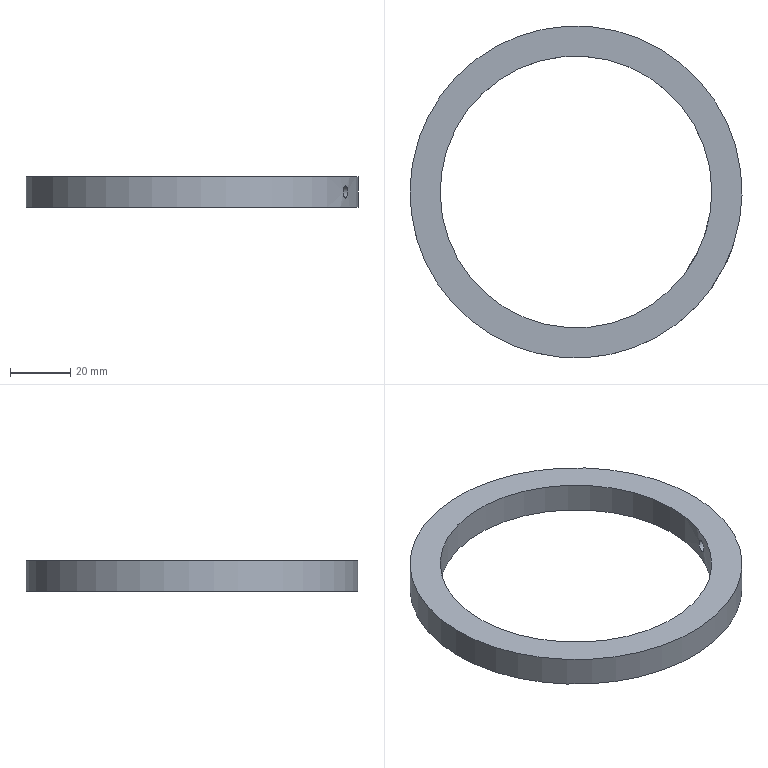Component | NX | CA6140-ZHUZHOU-ZHOUTAO3 | 1 solid | 5 faces | box 110 x 110 x 10 mm | volume 31291 mm3 | cylinder 3 | plane 2 | commonest cylinder face diameters 110 x1 90 x1 4 x1
STEP:
#1=CARTESIAN_POINT('',(0.,0.,0.));
#2=DIRECTION('',(0.,0.,1.));
#3=DIRECTION('',(1.,0.,0.));
#4=AXIS2_PLACEMENT_3D('',#1,#2,#3);
#5=CARTESIAN_POINT('',(17.204,41.581,-194.951));
#6=VERTEX_POINT('',#5);
#7=CARTESIAN_POINT('',(0.,-0.,-194.951));
#8=DIRECTION('',(0.,0.,-1.));
#9=DIRECTION('',(0.3823,0.924,0.));
#10=AXIS2_PLACEMENT_3D('',#7,#8,#9);
#11=CIRCLE('',#10,45.);
#12=CARTESIAN_POINT('',(0.,-0.,-194.951));
#13=DIRECTION('',(0.,0.,1.));
#14=DIRECTION('',(-0.3823,-0.924,0.));
#15=AXIS2_PLACEMENT_3D('',#12,#13,#14);
#16=PLANE('',#15);
#17=CARTESIAN_POINT('',(-45.,0.));
#18=CARTESIAN_POINT('',(-45.,77.942));
#19=CARTESIAN_POINT('',(22.5,38.971));
#20=CARTESIAN_POINT('',(90.,0.));
#21=CARTESIAN_POINT('',(22.5,-38.971));
#22=CARTESIAN_POINT('',(-45.,-77.942));
#23=CARTESIAN_POINT('',(-45.,0.));
#24=(BOUNDED_CURVE()B_SPLINE_CURVE(2,(#17,#18,#19,#20,#21,#22,#23),.UNSPECIFIED.,.T.,.F.)B_SPLINE_CURVE_WITH_KNOTS((1,2,2,2,2,1),(-2.094,0.,2.094,4.189,6.283,8.378),.UNSPECIFIED.)CURVE()GEOMETRIC_REPRESENTATION_ITEM()RATIONAL_B_SPLINE_CURVE((1.,0.5,1.,0.5,1.,0.5,1.))REPRESENTATION_ITEM(''));
#25=(GEOMETRIC_REPRESENTATION_CONTEXT(2)PARAMETRIC_REPRESENTATION_CONTEXT()REPRESENTATION_CONTEXT('',''));
#26=DEFINITIONAL_REPRESENTATION('',(#24),#25);
#27=PCURVE('',#16,#26);
#28=CARTESIAN_POINT('',(0.,-0.,-194.951));
#29=DIRECTION('',(0.,0.,-1.));
#30=DIRECTION('',(0.3823,0.924,0.));
#31=AXIS2_PLACEMENT_3D('',#28,#29,#30);
#32=CYLINDRICAL_SURFACE('',#31,45.);
#33=CARTESIAN_POINT('',(0.,0.));
#34=DIRECTION('',(1.,0.));
#35=VECTOR('',#34,1.);
#36=LINE('',#33,#35);
#37=(GEOMETRIC_REPRESENTATION_CONTEXT(2)PARAMETRIC_REPRESENTATION_CONTEXT()REPRESENTATION_CONTEXT('',''));
#38=DEFINITIONAL_REPRESENTATION('',(#36),#37);
#39=PCURVE('',#32,#38);
#40=SURFACE_CURVE('',#11,(#27,#39),.PCURVE_S1.);
#41=EDGE_CURVE('',#6,#6,#40,.T.);
#42=ORIENTED_EDGE('',*,*,#41,.T.);
#43=EDGE_LOOP('',(#42));
#44=FACE_BOUND('',#43,.T.);
#45=CARTESIAN_POINT('',(21.027,50.822,-194.951));
#46=VERTEX_POINT('',#45);
#47=CARTESIAN_POINT('',(-21.027,-50.822,-194.951));
#48=VERTEX_POINT('',#47);
#49=CARTESIAN_POINT('',(0.,-0.,-194.951));
#50=DIRECTION('',(0.,0.,-1.));
#51=DIRECTION('',(0.3823,0.924,0.));
#52=AXIS2_PLACEMENT_3D('',#49,#50,#51);
#53=CIRCLE('',#52,55.);
#54=CARTESIAN_POINT('',(-55.,0.));
#55=CARTESIAN_POINT('',(-55.,95.263));
#56=CARTESIAN_POINT('',(27.5,47.631));
#57=CARTESIAN_POINT('',(110.,0.));
#58=CARTESIAN_POINT('',(27.5,-47.631));
#59=CARTESIAN_POINT('',(-55.,-95.263));
#60=CARTESIAN_POINT('',(-55.,0.));
#61=(BOUNDED_CURVE()B_SPLINE_CURVE(2,(#54,#55,#56,#57,#58,#59,#60),.UNSPECIFIED.,.T.,.F.)B_SPLINE_CURVE_WITH_KNOTS((1,2,2,2,2,1),(-2.094,0.,2.094,4.189,6.283,8.378),.UNSPECIFIED.)CURVE()GEOMETRIC_REPRESENTATION_ITEM()RATIONAL_B_SPLINE_CURVE((1.,0.5,1.,0.5,1.,0.5,1.))REPRESENTATION_ITEM(''));
#62=(GEOMETRIC_REPRESENTATION_CONTEXT(2)PARAMETRIC_REPRESENTATION_CONTEXT()REPRESENTATION_CONTEXT('',''));
#63=DEFINITIONAL_REPRESENTATION('',(#61),#62);
#64=PCURVE('',#16,#63);
#65=CARTESIAN_POINT('',(0.,-0.,-204.951));
#66=DIRECTION('',(0.,0.,1.));
#67=DIRECTION('',(-0.3823,-0.924,0.));
#68=AXIS2_PLACEMENT_3D('',#65,#66,#67);
#69=CYLINDRICAL_SURFACE('',#68,55.);
#70=CARTESIAN_POINT('',(3.142,10.));
#71=DIRECTION('',(-1.,0.));
#72=VECTOR('',#71,1.);
#73=LINE('',#70,#72);
#74=(GEOMETRIC_REPRESENTATION_CONTEXT(2)PARAMETRIC_REPRESENTATION_CONTEXT()REPRESENTATION_CONTEXT('',''));
#75=DEFINITIONAL_REPRESENTATION('',(#73),#74);
#76=PCURVE('',#69,#75);
#77=SURFACE_CURVE('',#53,(#64,#76),.PCURVE_S1.);
#78=EDGE_CURVE('',#46,#48,#77,.T.);
#79=ORIENTED_EDGE('',*,*,#78,.F.);
#80=CARTESIAN_POINT('',(0.,-0.,-194.951));
#81=DIRECTION('',(0.,0.,-1.));
#82=DIRECTION('',(0.3823,0.924,0.));
#83=AXIS2_PLACEMENT_3D('',#80,#81,#82);
#84=CIRCLE('',#83,55.);
#85=CARTESIAN_POINT('',(-55.,0.));
#86=CARTESIAN_POINT('',(-55.,95.263));
#87=CARTESIAN_POINT('',(27.5,47.631));
#88=CARTESIAN_POINT('',(110.,0.));
#89=CARTESIAN_POINT('',(27.5,-47.631));
#90=CARTESIAN_POINT('',(-55.,-95.263));
#91=CARTESIAN_POINT('',(-55.,0.));
#92=(BOUNDED_CURVE()B_SPLINE_CURVE(2,(#85,#86,#87,#88,#89,#90,#91),.UNSPECIFIED.,.T.,.F.)B_SPLINE_CURVE_WITH_KNOTS((1,2,2,2,2,1),(-2.094,0.,2.094,4.189,6.283,8.378),.UNSPECIFIED.)CURVE()GEOMETRIC_REPRESENTATION_ITEM()RATIONAL_B_SPLINE_CURVE((1.,0.5,1.,0.5,1.,0.5,1.))REPRESENTATION_ITEM(''));
#93=(GEOMETRIC_REPRESENTATION_CONTEXT(2)PARAMETRIC_REPRESENTATION_CONTEXT()REPRESENTATION_CONTEXT('',''));
#94=DEFINITIONAL_REPRESENTATION('',(#92),#93);
#95=PCURVE('',#16,#94);
#96=CARTESIAN_POINT('',(9.425,10.));
#97=DIRECTION('',(-1.,0.));
#98=VECTOR('',#97,1.);
#99=LINE('',#96,#98);
#100=(GEOMETRIC_REPRESENTATION_CONTEXT(2)PARAMETRIC_REPRESENTATION_CONTEXT()REPRESENTATION_CONTEXT('',''));
#101=DEFINITIONAL_REPRESENTATION('',(#99),#100);
#102=PCURVE('',#69,#101);
#103=SURFACE_CURVE('',#84,(#95,#102),.PCURVE_S1.);
#104=EDGE_CURVE('',#48,#46,#103,.T.);
#105=ORIENTED_EDGE('',*,*,#104,.F.);
#106=EDGE_LOOP('',(#79,#105));
#107=FACE_BOUND('',#106,.T.);
#108=ADVANCED_FACE('',(#44,#107),#16,.T.);
#109=CARTESIAN_POINT('',(17.204,41.581,-204.951));
#110=VERTEX_POINT('',#109);
#111=CARTESIAN_POINT('',(0.,-0.,-204.951));
#112=DIRECTION('',(0.,0.,-1.));
#113=DIRECTION('',(0.3823,0.924,0.));
#114=AXIS2_PLACEMENT_3D('',#111,#112,#113);
#115=CIRCLE('',#114,45.);
#116=CARTESIAN_POINT('',(0.,-0.,-204.951));
#117=DIRECTION('',(0.,0.,-1.));
#118=DIRECTION('',(0.3823,0.924,0.));
#119=AXIS2_PLACEMENT_3D('',#116,#117,#118);
#120=PLANE('',#119);
#121=CARTESIAN_POINT('',(0.,0.));
#122=DIRECTION('',(1.,0.));
#123=AXIS2_PLACEMENT_2D('',#121,#122);
#124=CIRCLE('',#123,45.);
#125=(GEOMETRIC_REPRESENTATION_CONTEXT(2)PARAMETRIC_REPRESENTATION_CONTEXT()REPRESENTATION_CONTEXT('',''));
#126=DEFINITIONAL_REPRESENTATION('',(#124),#125);
#127=PCURVE('',#120,#126);
#128=CARTESIAN_POINT('',(0.,10.));
#129=DIRECTION('',(1.,0.));
#130=VECTOR('',#129,1.);
#131=LINE('',#128,#130);
#132=(GEOMETRIC_REPRESENTATION_CONTEXT(2)PARAMETRIC_REPRESENTATION_CONTEXT()REPRESENTATION_CONTEXT('',''));
#133=DEFINITIONAL_REPRESENTATION('',(#131),#132);
#134=PCURVE('',#32,#133);
#135=SURFACE_CURVE('',#115,(#127,#134),.PCURVE_S1.);
#136=EDGE_CURVE('',#110,#110,#135,.T.);
#137=ORIENTED_EDGE('',*,*,#136,.F.);
#138=EDGE_LOOP('',(#137));
#139=FACE_BOUND('',#138,.T.);
#140=CARTESIAN_POINT('',(-21.027,-50.822,-204.951));
#141=VERTEX_POINT('',#140);
#142=CARTESIAN_POINT('',(0.,-0.,-204.951));
#143=DIRECTION('',(0.,0.,1.));
#144=DIRECTION('',(-0.3823,-0.924,0.));
#145=AXIS2_PLACEMENT_3D('',#142,#143,#144);
#146=CIRCLE('',#145,55.);
#147=CARTESIAN_POINT('',(-55.,0.));
#148=CARTESIAN_POINT('',(-55.,95.263));
#149=CARTESIAN_POINT('',(27.5,47.631));
#150=CARTESIAN_POINT('',(110.,0.));
#151=CARTESIAN_POINT('',(27.5,-47.631));
#152=CARTESIAN_POINT('',(-55.,-95.263));
#153=CARTESIAN_POINT('',(-55.,0.));
#154=(BOUNDED_CURVE()B_SPLINE_CURVE(2,(#147,#148,#149,#150,#151,#152,#153),.UNSPECIFIED.,.T.,.F.)B_SPLINE_CURVE_WITH_KNOTS((1,2,2,2,2,1),(-2.094,0.,2.094,4.189,6.283,8.378),.UNSPECIFIED.)CURVE()GEOMETRIC_REPRESENTATION_ITEM()RATIONAL_B_SPLINE_CURVE((1.,0.5,1.,0.5,1.,0.5,1.))REPRESENTATION_ITEM(''));
#155=(GEOMETRIC_REPRESENTATION_CONTEXT(2)PARAMETRIC_REPRESENTATION_CONTEXT()REPRESENTATION_CONTEXT('',''));
#156=DEFINITIONAL_REPRESENTATION('',(#154),#155);
#157=PCURVE('',#120,#156);
#158=CARTESIAN_POINT('',(0.,0.));
#159=DIRECTION('',(1.,0.));
#160=VECTOR('',#159,1.);
#161=LINE('',#158,#160);
#162=(GEOMETRIC_REPRESENTATION_CONTEXT(2)PARAMETRIC_REPRESENTATION_CONTEXT()REPRESENTATION_CONTEXT('',''));
#163=DEFINITIONAL_REPRESENTATION('',(#161),#162);
#164=PCURVE('',#69,#163);
#165=SURFACE_CURVE('',#146,(#157,#164),.PCURVE_S1.);
#166=EDGE_CURVE('',#141,#141,#165,.T.);
#167=ORIENTED_EDGE('',*,*,#166,.F.);
#168=EDGE_LOOP('',(#167));
#169=FACE_BOUND('',#168,.T.);
#170=ADVANCED_FACE('',(#139,#169),#120,.T.);
#171=ORIENTED_EDGE('',*,*,#78,.T.);
#172=CARTESIAN_POINT('',(-21.027,-50.822,-204.951));
#173=CARTESIAN_POINT('',(-21.027,-50.822,-194.951));
#174=B_SPLINE_CURVE_WITH_KNOTS('',1,(#172,#173),.UNSPECIFIED.,.F.,.F.,(2,2),(0.,10.),.PIECEWISE_BEZIER_KNOTS.);
#175=CARTESIAN_POINT('',(0.,0.));
#176=DIRECTION('',(0.,1.));
#177=VECTOR('',#176,1.);
#178=LINE('',#175,#177);
#179=(GEOMETRIC_REPRESENTATION_CONTEXT(2)PARAMETRIC_REPRESENTATION_CONTEXT()REPRESENTATION_CONTEXT('',''));
#180=DEFINITIONAL_REPRESENTATION('',(#178),#179);
#181=PCURVE('',#69,#180);
#182=CARTESIAN_POINT('',(6.283,0.));
#183=DIRECTION('',(0.,1.));
#184=VECTOR('',#183,1.);
#185=LINE('',#182,#184);
#186=(GEOMETRIC_REPRESENTATION_CONTEXT(2)PARAMETRIC_REPRESENTATION_CONTEXT()REPRESENTATION_CONTEXT('',''));
#187=DEFINITIONAL_REPRESENTATION('',(#185),#186);
#188=PCURVE('',#69,#187);
#189=SEAM_CURVE('',#174,(#181,#188),.PCURVE_S1.);
#190=EDGE_CURVE('',#141,#48,#189,.T.);
#191=ORIENTED_EDGE('',*,*,#190,.F.);
#192=ORIENTED_EDGE('',*,*,#166,.T.);
#193=ORIENTED_EDGE('',*,*,#190,.T.);
#194=ORIENTED_EDGE('',*,*,#104,.T.);
#195=EDGE_LOOP('',(#171,#191,#192,#193,#194));
#196=FACE_BOUND('',#195,.T.);
#197=CARTESIAN_POINT('',(50.822,-21.027,-201.951));
#198=VERTEX_POINT('',#197);
#199=CARTESIAN_POINT('',(50.822,-21.027,-201.951));
#200=CARTESIAN_POINT('',(50.907,-20.821,-201.951));
#201=CARTESIAN_POINT('',(50.993,-20.611,-201.912));
#202=CARTESIAN_POINT('',(51.071,-20.414,-201.838));
#203=CARTESIAN_POINT('',(51.149,-20.218,-201.764));
#204=CARTESIAN_POINT('',(51.223,-20.031,-201.653));
#205=CARTESIAN_POINT('',(51.286,-19.868,-201.513));
#206=CARTESIAN_POINT('',(51.349,-19.705,-201.373));
#207=CARTESIAN_POINT('',(51.404,-19.562,-201.201));
#208=CARTESIAN_POINT('',(51.446,-19.451,-201.011));
#209=CARTESIAN_POINT('',(51.488,-19.34,-200.822));
#210=CARTESIAN_POINT('',(51.518,-19.258,-200.609));
#211=CARTESIAN_POINT('',(51.536,-19.211,-200.39));
#212=CARTESIAN_POINT('',(51.553,-19.165,-200.172));
#213=CARTESIAN_POINT('',(51.557,-19.154,-199.942));
#214=CARTESIAN_POINT('',(51.548,-19.178,-199.72));
#215=CARTESIAN_POINT('',(51.539,-19.202,-199.498));
#216=CARTESIAN_POINT('',(51.517,-19.263,-199.277));
#217=CARTESIAN_POINT('',(51.482,-19.354,-199.076));
#218=CARTESIAN_POINT('',(51.448,-19.446,-198.874));
#219=CARTESIAN_POINT('',(51.4,-19.572,-198.687));
#220=CARTESIAN_POINT('',(51.343,-19.72,-198.53));
#221=CARTESIAN_POINT('',(51.286,-19.868,-198.372));
#222=CARTESIAN_POINT('',(51.218,-20.044,-198.24));
#223=CARTESIAN_POINT('',(51.144,-20.232,-198.144));
#224=CARTESIAN_POINT('',(51.069,-20.42,-198.048));
#225=CARTESIAN_POINT('',(50.986,-20.626,-197.986));
#226=CARTESIAN_POINT('',(50.902,-20.832,-197.962));
#227=CARTESIAN_POINT('',(50.818,-21.038,-197.938));
#228=CARTESIAN_POINT('',(50.73,-21.25,-197.953));
#229=CARTESIAN_POINT('',(50.645,-21.45,-198.004));
#230=CARTESIAN_POINT('',(50.56,-21.651,-198.055));
#231=CARTESIAN_POINT('',(50.476,-21.846,-198.145));
#232=CARTESIAN_POINT('',(50.4,-22.018,-198.265));
#233=CARTESIAN_POINT('',(50.325,-22.191,-198.386));
#234=CARTESIAN_POINT('',(50.256,-22.347,-198.54));
#235=CARTESIAN_POINT('',(50.199,-22.473,-198.716));
#236=CARTESIAN_POINT('',(50.143,-22.599,-198.893));
#237=CARTESIAN_POINT('',(50.097,-22.699,-199.095));
#238=CARTESIAN_POINT('',(50.068,-22.765,-199.307));
#239=CARTESIAN_POINT('',(50.038,-22.83,-199.519));
#240=CARTESIAN_POINT('',(50.023,-22.864,-199.746));
#241=CARTESIAN_POINT('',(50.023,-22.862,-199.97));
#242=CARTESIAN_POINT('',(50.024,-22.86,-200.194));
#243=CARTESIAN_POINT('',(50.041,-22.822,-200.42));
#244=CARTESIAN_POINT('',(50.073,-22.753,-200.631));
#245=CARTESIAN_POINT('',(50.104,-22.684,-200.841));
#246=CARTESIAN_POINT('',(50.151,-22.58,-201.041));
#247=CARTESIAN_POINT('',(50.209,-22.451,-201.215));
#248=CARTESIAN_POINT('',(50.267,-22.322,-201.388));
#249=CARTESIAN_POINT('',(50.337,-22.164,-201.54));
#250=CARTESIAN_POINT('',(50.413,-21.989,-201.656));
#251=CARTESIAN_POINT('',(50.49,-21.814,-201.773));
#252=CARTESIAN_POINT('',(50.574,-21.617,-201.859));
#253=CARTESIAN_POINT('',(50.659,-21.416,-201.906));
#254=CARTESIAN_POINT('',(50.713,-21.289,-201.936));
#255=CARTESIAN_POINT('',(50.768,-21.158,-201.951));
#256=CARTESIAN_POINT('',(50.822,-21.027,-201.951));
#257=B_SPLINE_CURVE_WITH_KNOTS('',3,(#199,#200,#201,#202,#203,#204,#205,#206,#207,#208,#209,#210,#211,#212,#213,#214,#215,#216,#217,#218,#219,#220,#221,#222,#223,#224,#225,#226,#227,#228,#229,#230,#231,#232,#233,#234,#235,#236,#237,#238,#239,#240,#241,#242,#243,#244,#245,#246,#247,#248,#249,#250,#251,#252,#253,#254,#255,#256),.UNSPECIFIED.,.T.,.F.,(1,3,3,3,3,3,3,3,3,3,3,3,3,3,3,3,3,3,3,3,3,1),(-0.03354,0.,0.05368,0.1074,0.1611,0.2148,0.2685,0.3221,0.3758,0.4295,0.4832,0.5369,0.5906,0.6443,0.698,0.7517,0.8054,0.859,0.9127,0.9665,1.,1.054),.UNSPECIFIED.);
#258=CARTESIAN_POINT('',(1.571,3.));
#259=CARTESIAN_POINT('',(1.572,3.));
#260=CARTESIAN_POINT('',(1.573,3.003));
#261=CARTESIAN_POINT('',(1.576,3.019));
#262=CARTESIAN_POINT('',(1.579,3.044));
#263=CARTESIAN_POINT('',(1.581,3.08));
#264=CARTESIAN_POINT('',(1.584,3.124));
#265=CARTESIAN_POINT('',(1.586,3.179));
#266=CARTESIAN_POINT('',(1.588,3.243));
#267=CARTESIAN_POINT('',(1.59,3.316));
#268=CARTESIAN_POINT('',(1.593,3.398));
#269=CARTESIAN_POINT('',(1.595,3.487));
#270=CARTESIAN_POINT('',(1.597,3.584));
#271=CARTESIAN_POINT('',(1.598,3.689));
#272=CARTESIAN_POINT('',(1.6,3.801));
#273=CARTESIAN_POINT('',(1.601,3.918));
#274=CARTESIAN_POINT('',(1.603,4.04));
#275=CARTESIAN_POINT('',(1.604,4.168));
#276=CARTESIAN_POINT('',(1.605,4.3));
#277=CARTESIAN_POINT('',(1.606,4.436));
#278=CARTESIAN_POINT('',(1.606,4.574));
#279=CARTESIAN_POINT('',(1.607,4.714));
#280=CARTESIAN_POINT('',(1.607,4.857));
#281=CARTESIAN_POINT('',(1.607,5.));
#282=CARTESIAN_POINT('',(1.607,5.143));
#283=CARTESIAN_POINT('',(1.607,5.284));
#284=CARTESIAN_POINT('',(1.606,5.424));
#285=CARTESIAN_POINT('',(1.606,5.563));
#286=CARTESIAN_POINT('',(1.605,5.699));
#287=CARTESIAN_POINT('',(1.604,5.831));
#288=CARTESIAN_POINT('',(1.603,5.958));
#289=CARTESIAN_POINT('',(1.601,6.081));
#290=CARTESIAN_POINT('',(1.6,6.199));
#291=CARTESIAN_POINT('',(1.598,6.31));
#292=CARTESIAN_POINT('',(1.597,6.415));
#293=CARTESIAN_POINT('',(1.595,6.512));
#294=CARTESIAN_POINT('',(1.593,6.602));
#295=CARTESIAN_POINT('',(1.59,6.683));
#296=CARTESIAN_POINT('',(1.588,6.757));
#297=CARTESIAN_POINT('',(1.586,6.82));
#298=CARTESIAN_POINT('',(1.584,6.875));
#299=CARTESIAN_POINT('',(1.581,6.92));
#300=CARTESIAN_POINT('',(1.579,6.956));
#301=CARTESIAN_POINT('',(1.576,6.981));
#302=CARTESIAN_POINT('',(1.573,6.996));
#303=CARTESIAN_POINT('',(1.571,7.002));
#304=CARTESIAN_POINT('',(1.568,6.996));
#305=CARTESIAN_POINT('',(1.566,6.981));
#306=CARTESIAN_POINT('',(1.563,6.956));
#307=CARTESIAN_POINT('',(1.561,6.921));
#308=CARTESIAN_POINT('',(1.558,6.876));
#309=CARTESIAN_POINT('',(1.556,6.821));
#310=CARTESIAN_POINT('',(1.553,6.757));
#311=CARTESIAN_POINT('',(1.551,6.685));
#312=CARTESIAN_POINT('',(1.549,6.603));
#313=CARTESIAN_POINT('',(1.547,6.514));
#314=CARTESIAN_POINT('',(1.545,6.416));
#315=CARTESIAN_POINT('',(1.543,6.312));
#316=CARTESIAN_POINT('',(1.542,6.201));
#317=CARTESIAN_POINT('',(1.54,6.084));
#318=CARTESIAN_POINT('',(1.539,5.961));
#319=CARTESIAN_POINT('',(1.538,5.833));
#320=CARTESIAN_POINT('',(1.537,5.701));
#321=CARTESIAN_POINT('',(1.536,5.566));
#322=CARTESIAN_POINT('',(1.535,5.427));
#323=CARTESIAN_POINT('',(1.535,5.287));
#324=CARTESIAN_POINT('',(1.534,5.144));
#325=CARTESIAN_POINT('',(1.534,5.002));
#326=CARTESIAN_POINT('',(1.534,4.86));
#327=CARTESIAN_POINT('',(1.535,4.717));
#328=CARTESIAN_POINT('',(1.535,4.576));
#329=CARTESIAN_POINT('',(1.536,4.437));
#330=CARTESIAN_POINT('',(1.537,4.302));
#331=CARTESIAN_POINT('',(1.538,4.171));
#332=CARTESIAN_POINT('',(1.539,4.043));
#333=CARTESIAN_POINT('',(1.54,3.919));
#334=CARTESIAN_POINT('',(1.542,3.802));
#335=CARTESIAN_POINT('',(1.543,3.691));
#336=CARTESIAN_POINT('',(1.545,3.586));
#337=CARTESIAN_POINT('',(1.547,3.489));
#338=CARTESIAN_POINT('',(1.549,3.399));
#339=CARTESIAN_POINT('',(1.551,3.317));
#340=CARTESIAN_POINT('',(1.553,3.244));
#341=CARTESIAN_POINT('',(1.556,3.18));
#342=CARTESIAN_POINT('',(1.558,3.125));
#343=CARTESIAN_POINT('',(1.561,3.08));
#344=CARTESIAN_POINT('',(1.563,3.045));
#345=CARTESIAN_POINT('',(1.566,3.019));
#346=CARTESIAN_POINT('',(1.568,3.003));
#347=CARTESIAN_POINT('',(1.57,3.));
#348=CARTESIAN_POINT('',(1.571,3.));
#349=B_SPLINE_CURVE_WITH_KNOTS('',3,(#258,#259,#260,#261,#262,#263,#264,#265,#266,#267,#268,#269,#270,#271,#272,#273,#274,#275,#276,#277,#278,#279,#280,#281,#282,#283,#284,#285,#286,#287,#288,#289,#290,#291,#292,#293,#294,#295,#296,#297,#298,#299,#300,#301,#302,#303,#304,#305,#306,#307,#308,#309,#310,#311,#312,#313,#314,#315,#316,#317,#318,#319,#320,#321,#322,#323,#324,#325,#326,#327,#328,#329,#330,#331,#332,#333,#334,#335,#336,#337,#338,#339,#340,#341,#342,#343,#344,#345,#346,#347,#348),.UNSPECIFIED.,.T.,.F.,(4,1,1,1,1,1,1,1,1,1,1,1,1,1,1,1,1,1,1,1,1,1,1,1,1,1,1,1,1,1,1,1,1,1,1,1,1,1,1,1,1,1,1,1,1,1,1,1,1,1,1,1,1,1,1,1,1,1,1,1,1,1,1,1,1,1,1,1,1,1,1,1,1,1,1,1,1,1,1,1,1,1,1,1,1,1,1,1,4),(0.,0.01136,0.02273,0.03409,0.04545,0.05682,0.06818,0.07955,0.09091,0.1023,0.1136,0.125,0.1364,0.1477,0.1591,0.1705,0.1818,0.1932,0.2045,0.2159,0.2273,0.2386,0.25,0.2614,0.2727,0.2841,0.2955,0.3068,0.3182,0.3295,0.3409,0.3523,0.3636,0.375,0.3864,0.3977,0.4091,0.4205,0.4318,0.4432,0.4545,0.4659,0.4773,0.4886,0.5,0.5114,0.5227,0.5341,0.5455,0.5568,0.5682,0.5795,0.5909,0.6023,0.6136,0.625,0.6364,0.6477,0.6591,0.6705,0.6818,0.6932,0.7045,0.7159,0.7273,0.7386,0.75,0.7614,0.7727,0.7841,0.7955,0.8068,0.8182,0.8295,0.8409,0.8523,0.8636,0.875,0.8864,0.8977,0.9091,0.9205,0.9318,0.9432,0.9545,0.9659,0.9773,0.9886,1.),.QUASI_UNIFORM_KNOTS.);
#350=(GEOMETRIC_REPRESENTATION_CONTEXT(2)PARAMETRIC_REPRESENTATION_CONTEXT()REPRESENTATION_CONTEXT('',''));
#351=DEFINITIONAL_REPRESENTATION('',(#349),#350);
#352=PCURVE('',#69,#351);
#353=CARTESIAN_POINT('',(55.442,-22.939,-199.951));
#354=DIRECTION('',(-0.924,0.3823,0.));
#355=DIRECTION('',(0.,0.,-1.));
#356=AXIS2_PLACEMENT_3D('',#353,#354,#355);
#357=CYLINDRICAL_SURFACE('',#356,2.);
#358=CARTESIAN_POINT('',(6.283,5.));
#359=CARTESIAN_POINT('',(0.,5.));
#360=B_SPLINE_CURVE_WITH_KNOTS('',1,(#358,#359),.UNSPECIFIED.,.F.,.F.,(2,2),(0.,1.),.PIECEWISE_BEZIER_KNOTS.);
#361=(GEOMETRIC_REPRESENTATION_CONTEXT(2)PARAMETRIC_REPRESENTATION_CONTEXT()REPRESENTATION_CONTEXT('',''));
#362=DEFINITIONAL_REPRESENTATION('',(#360),#361);
#363=PCURVE('',#357,#362);
#364=SURFACE_CURVE('',#257,(#352,#363),.PCURVE_S1.);
#365=EDGE_CURVE('',#198,#198,#364,.T.);
#366=ORIENTED_EDGE('',*,*,#365,.F.);
#367=EDGE_LOOP('',(#366));
#368=FACE_BOUND('',#367,.T.);
#369=ADVANCED_FACE('',(#196,#368),#69,.T.);
#370=ORIENTED_EDGE('',*,*,#136,.F.);
#371=CARTESIAN_POINT('',(17.204,41.581,-194.951));
#372=CARTESIAN_POINT('',(17.204,41.581,-204.951));
#373=B_SPLINE_CURVE_WITH_KNOTS('',1,(#371,#372),.UNSPECIFIED.,.F.,.F.,(2,2),(0.,10.),.PIECEWISE_BEZIER_KNOTS.);
#374=CARTESIAN_POINT('',(0.,0.));
#375=DIRECTION('',(0.,1.));
#376=VECTOR('',#375,1.);
#377=LINE('',#374,#376);
#378=(GEOMETRIC_REPRESENTATION_CONTEXT(2)PARAMETRIC_REPRESENTATION_CONTEXT()REPRESENTATION_CONTEXT('',''));
#379=DEFINITIONAL_REPRESENTATION('',(#377),#378);
#380=PCURVE('',#32,#379);
#381=CARTESIAN_POINT('',(6.283,0.));
#382=DIRECTION('',(0.,1.));
#383=VECTOR('',#382,1.);
#384=LINE('',#381,#383);
#385=(GEOMETRIC_REPRESENTATION_CONTEXT(2)PARAMETRIC_REPRESENTATION_CONTEXT()REPRESENTATION_CONTEXT('',''));
#386=DEFINITIONAL_REPRESENTATION('',(#384),#385);
#387=PCURVE('',#32,#386);
#388=SEAM_CURVE('',#373,(#380,#387),.PCURVE_S1.);
#389=EDGE_CURVE('',#6,#110,#388,.T.);
#390=ORIENTED_EDGE('',*,*,#389,.F.);
#391=ORIENTED_EDGE('',*,*,#41,.T.);
#392=ORIENTED_EDGE('',*,*,#389,.T.);
#393=EDGE_LOOP('',(#370,#390,#391,#392));
#394=FACE_BOUND('',#393,.F.);
#395=CARTESIAN_POINT('',(41.581,-17.204,-201.951));
#396=VERTEX_POINT('',#395);
#397=CARTESIAN_POINT('',(41.581,-17.204,-201.951));
#398=CARTESIAN_POINT('',(41.667,-16.998,-201.951));
#399=CARTESIAN_POINT('',(41.752,-16.787,-201.912));
#400=CARTESIAN_POINT('',(41.83,-16.591,-201.838));
#401=CARTESIAN_POINT('',(41.908,-16.395,-201.764));
#402=CARTESIAN_POINT('',(41.98,-16.207,-201.653));
#403=CARTESIAN_POINT('',(42.043,-16.044,-201.513));
#404=CARTESIAN_POINT('',(42.105,-15.88,-201.373));
#405=CARTESIAN_POINT('',(42.159,-15.737,-201.201));
#406=CARTESIAN_POINT('',(42.2,-15.626,-201.012));
#407=CARTESIAN_POINT('',(42.241,-15.514,-200.822));
#408=CARTESIAN_POINT('',(42.271,-15.432,-200.609));
#409=CARTESIAN_POINT('',(42.288,-15.385,-200.391));
#410=CARTESIAN_POINT('',(42.305,-15.339,-200.172));
#411=CARTESIAN_POINT('',(42.309,-15.328,-199.942));
#412=CARTESIAN_POINT('',(42.3,-15.352,-199.72));
#413=CARTESIAN_POINT('',(42.292,-15.376,-199.498));
#414=CARTESIAN_POINT('',(42.27,-15.437,-199.277));
#415=CARTESIAN_POINT('',(42.236,-15.529,-199.076));
#416=CARTESIAN_POINT('',(42.202,-15.62,-198.875));
#417=CARTESIAN_POINT('',(42.156,-15.746,-198.688));
#418=CARTESIAN_POINT('',(42.099,-15.895,-198.53));
#419=CARTESIAN_POINT('',(42.043,-16.044,-198.373));
#420=CARTESIAN_POINT('',(41.976,-16.22,-198.24));
#421=CARTESIAN_POINT('',(41.902,-16.408,-198.144));
#422=CARTESIAN_POINT('',(41.828,-16.596,-198.048));
#423=CARTESIAN_POINT('',(41.746,-16.802,-197.986));
#424=CARTESIAN_POINT('',(41.662,-17.008,-197.962));
#425=CARTESIAN_POINT('',(41.578,-17.214,-197.938));
#426=CARTESIAN_POINT('',(41.49,-17.426,-197.953));
#427=CARTESIAN_POINT('',(41.404,-17.626,-198.004));
#428=CARTESIAN_POINT('',(41.319,-17.827,-198.055));
#429=CARTESIAN_POINT('',(41.234,-18.021,-198.144));
#430=CARTESIAN_POINT('',(41.158,-18.193,-198.265));
#431=CARTESIAN_POINT('',(41.082,-18.366,-198.385));
#432=CARTESIAN_POINT('',(41.012,-18.522,-198.54));
#433=CARTESIAN_POINT('',(40.955,-18.647,-198.716));
#434=CARTESIAN_POINT('',(40.897,-18.773,-198.892));
#435=CARTESIAN_POINT('',(40.851,-18.873,-199.094));
#436=CARTESIAN_POINT('',(40.821,-18.939,-199.306));
#437=CARTESIAN_POINT('',(40.79,-19.004,-199.518));
#438=CARTESIAN_POINT('',(40.775,-19.037,-199.745));
#439=CARTESIAN_POINT('',(40.776,-19.035,-199.969));
#440=CARTESIAN_POINT('',(40.777,-19.033,-200.193));
#441=CARTESIAN_POINT('',(40.794,-18.997,-200.419));
#442=CARTESIAN_POINT('',(40.826,-18.928,-200.63));
#443=CARTESIAN_POINT('',(40.858,-18.859,-200.84));
#444=CARTESIAN_POINT('',(40.905,-18.756,-201.04));
#445=CARTESIAN_POINT('',(40.964,-18.627,-201.214));
#446=CARTESIAN_POINT('',(41.022,-18.498,-201.387));
#447=CARTESIAN_POINT('',(41.093,-18.34,-201.539));
#448=CARTESIAN_POINT('',(41.17,-18.166,-201.656));
#449=CARTESIAN_POINT('',(41.247,-17.991,-201.773));
#450=CARTESIAN_POINT('',(41.333,-17.795,-201.858));
#451=CARTESIAN_POINT('',(41.418,-17.594,-201.906));
#452=CARTESIAN_POINT('',(41.472,-17.466,-201.936));
#453=CARTESIAN_POINT('',(41.527,-17.335,-201.951));
#454=CARTESIAN_POINT('',(41.581,-17.204,-201.951));
#455=B_SPLINE_CURVE_WITH_KNOTS('',3,(#397,#398,#399,#400,#401,#402,#403,#404,#405,#406,#407,#408,#409,#410,#411,#412,#413,#414,#415,#416,#417,#418,#419,#420,#421,#422,#423,#424,#425,#426,#427,#428,#429,#430,#431,#432,#433,#434,#435,#436,#437,#438,#439,#440,#441,#442,#443,#444,#445,#446,#447,#448,#449,#450,#451,#452,#453,#454),.UNSPECIFIED.,.T.,.F.,(1,3,3,3,3,3,3,3,3,3,3,3,3,3,3,3,3,3,3,3,3,1),(-0.03365,0.,0.05367,0.1073,0.161,0.2148,0.2684,0.3221,0.3758,0.4295,0.4832,0.5369,0.5905,0.6442,0.6979,0.7516,0.8053,0.8589,0.9126,0.9663,1.,1.054),.UNSPECIFIED.);
#456=CARTESIAN_POINT('',(1.571,7.));
#457=CARTESIAN_POINT('',(1.57,7.));
#458=CARTESIAN_POINT('',(1.568,6.997));
#459=CARTESIAN_POINT('',(1.564,6.981));
#460=CARTESIAN_POINT('',(1.561,6.956));
#461=CARTESIAN_POINT('',(1.558,6.92));
#462=CARTESIAN_POINT('',(1.555,6.876));
#463=CARTESIAN_POINT('',(1.552,6.821));
#464=CARTESIAN_POINT('',(1.549,6.757));
#465=CARTESIAN_POINT('',(1.547,6.684));
#466=CARTESIAN_POINT('',(1.544,6.602));
#467=CARTESIAN_POINT('',(1.542,6.513));
#468=CARTESIAN_POINT('',(1.539,6.416));
#469=CARTESIAN_POINT('',(1.537,6.311));
#470=CARTESIAN_POINT('',(1.535,6.199));
#471=CARTESIAN_POINT('',(1.533,6.082));
#472=CARTESIAN_POINT('',(1.532,5.96));
#473=CARTESIAN_POINT('',(1.53,5.832));
#474=CARTESIAN_POINT('',(1.529,5.7));
#475=CARTESIAN_POINT('',(1.528,5.564));
#476=CARTESIAN_POINT('',(1.527,5.426));
#477=CARTESIAN_POINT('',(1.527,5.286));
#478=CARTESIAN_POINT('',(1.526,5.143));
#479=CARTESIAN_POINT('',(1.526,5.));
#480=CARTESIAN_POINT('',(1.526,4.857));
#481=CARTESIAN_POINT('',(1.527,4.716));
#482=CARTESIAN_POINT('',(1.527,4.576));
#483=CARTESIAN_POINT('',(1.528,4.437));
#484=CARTESIAN_POINT('',(1.529,4.301));
#485=CARTESIAN_POINT('',(1.53,4.169));
#486=CARTESIAN_POINT('',(1.532,4.042));
#487=CARTESIAN_POINT('',(1.533,3.919));
#488=CARTESIAN_POINT('',(1.535,3.801));
#489=CARTESIAN_POINT('',(1.537,3.69));
#490=CARTESIAN_POINT('',(1.539,3.585));
#491=CARTESIAN_POINT('',(1.542,3.488));
#492=CARTESIAN_POINT('',(1.544,3.398));
#493=CARTESIAN_POINT('',(1.547,3.317));
#494=CARTESIAN_POINT('',(1.549,3.244));
#495=CARTESIAN_POINT('',(1.552,3.18));
#496=CARTESIAN_POINT('',(1.555,3.125));
#497=CARTESIAN_POINT('',(1.558,3.08));
#498=CARTESIAN_POINT('',(1.561,3.044));
#499=CARTESIAN_POINT('',(1.564,3.019));
#500=CARTESIAN_POINT('',(1.568,3.004));
#501=CARTESIAN_POINT('',(1.571,2.998));
#502=CARTESIAN_POINT('',(1.574,3.004));
#503=CARTESIAN_POINT('',(1.577,3.019));
#504=CARTESIAN_POINT('',(1.58,3.044));
#505=CARTESIAN_POINT('',(1.583,3.079));
#506=CARTESIAN_POINT('',(1.586,3.124));
#507=CARTESIAN_POINT('',(1.589,3.179));
#508=CARTESIAN_POINT('',(1.592,3.243));
#509=CARTESIAN_POINT('',(1.595,3.315));
#510=CARTESIAN_POINT('',(1.597,3.397));
#511=CARTESIAN_POINT('',(1.6,3.486));
#512=CARTESIAN_POINT('',(1.602,3.584));
#513=CARTESIAN_POINT('',(1.604,3.688));
#514=CARTESIAN_POINT('',(1.606,3.799));
#515=CARTESIAN_POINT('',(1.608,3.916));
#516=CARTESIAN_POINT('',(1.61,4.039));
#517=CARTESIAN_POINT('',(1.611,4.167));
#518=CARTESIAN_POINT('',(1.612,4.299));
#519=CARTESIAN_POINT('',(1.613,4.434));
#520=CARTESIAN_POINT('',(1.614,4.573));
#521=CARTESIAN_POINT('',(1.615,4.713));
#522=CARTESIAN_POINT('',(1.615,4.856));
#523=CARTESIAN_POINT('',(1.615,4.998));
#524=CARTESIAN_POINT('',(1.615,5.141));
#525=CARTESIAN_POINT('',(1.615,5.283));
#526=CARTESIAN_POINT('',(1.614,5.424));
#527=CARTESIAN_POINT('',(1.613,5.563));
#528=CARTESIAN_POINT('',(1.613,5.698));
#529=CARTESIAN_POINT('',(1.611,5.829));
#530=CARTESIAN_POINT('',(1.61,5.957));
#531=CARTESIAN_POINT('',(1.608,6.081));
#532=CARTESIAN_POINT('',(1.606,6.198));
#533=CARTESIAN_POINT('',(1.604,6.309));
#534=CARTESIAN_POINT('',(1.602,6.414));
#535=CARTESIAN_POINT('',(1.6,6.511));
#536=CARTESIAN_POINT('',(1.597,6.601));
#537=CARTESIAN_POINT('',(1.595,6.683));
#538=CARTESIAN_POINT('',(1.592,6.755));
#539=CARTESIAN_POINT('',(1.589,6.82));
#540=CARTESIAN_POINT('',(1.586,6.875));
#541=CARTESIAN_POINT('',(1.583,6.92));
#542=CARTESIAN_POINT('',(1.58,6.955));
#543=CARTESIAN_POINT('',(1.577,6.981));
#544=CARTESIAN_POINT('',(1.574,6.997));
#545=CARTESIAN_POINT('',(1.572,7.));
#546=CARTESIAN_POINT('',(1.571,7.));
#547=B_SPLINE_CURVE_WITH_KNOTS('',3,(#456,#457,#458,#459,#460,#461,#462,#463,#464,#465,#466,#467,#468,#469,#470,#471,#472,#473,#474,#475,#476,#477,#478,#479,#480,#481,#482,#483,#484,#485,#486,#487,#488,#489,#490,#491,#492,#493,#494,#495,#496,#497,#498,#499,#500,#501,#502,#503,#504,#505,#506,#507,#508,#509,#510,#511,#512,#513,#514,#515,#516,#517,#518,#519,#520,#521,#522,#523,#524,#525,#526,#527,#528,#529,#530,#531,#532,#533,#534,#535,#536,#537,#538,#539,#540,#541,#542,#543,#544,#545,#546),.UNSPECIFIED.,.T.,.F.,(4,1,1,1,1,1,1,1,1,1,1,1,1,1,1,1,1,1,1,1,1,1,1,1,1,1,1,1,1,1,1,1,1,1,1,1,1,1,1,1,1,1,1,1,1,1,1,1,1,1,1,1,1,1,1,1,1,1,1,1,1,1,1,1,1,1,1,1,1,1,1,1,1,1,1,1,1,1,1,1,1,1,1,1,1,1,1,1,4),(0.,0.01136,0.02273,0.03409,0.04545,0.05682,0.06818,0.07955,0.09091,0.1023,0.1136,0.125,0.1364,0.1477,0.1591,0.1705,0.1818,0.1932,0.2045,0.2159,0.2273,0.2386,0.25,0.2614,0.2727,0.2841,0.2955,0.3068,0.3182,0.3295,0.3409,0.3523,0.3636,0.375,0.3864,0.3977,0.4091,0.4205,0.4318,0.4432,0.4545,0.4659,0.4773,0.4886,0.5,0.5114,0.5227,0.5341,0.5455,0.5568,0.5682,0.5795,0.5909,0.6023,0.6136,0.625,0.6364,0.6477,0.6591,0.6705,0.6818,0.6932,0.7045,0.7159,0.7273,0.7386,0.75,0.7614,0.7727,0.7841,0.7955,0.8068,0.8182,0.8295,0.8409,0.8523,0.8636,0.875,0.8864,0.8977,0.9091,0.9205,0.9318,0.9432,0.9545,0.9659,0.9773,0.9886,1.),.QUASI_UNIFORM_KNOTS.);
#548=(GEOMETRIC_REPRESENTATION_CONTEXT(2)PARAMETRIC_REPRESENTATION_CONTEXT()REPRESENTATION_CONTEXT('',''));
#549=DEFINITIONAL_REPRESENTATION('',(#547),#548);
#550=PCURVE('',#32,#549);
#551=CARTESIAN_POINT('',(6.283,15.));
#552=CARTESIAN_POINT('',(0.,15.));
#553=B_SPLINE_CURVE_WITH_KNOTS('',1,(#551,#552),.UNSPECIFIED.,.F.,.F.,(2,2),(0.,1.),.PIECEWISE_BEZIER_KNOTS.);
#554=(GEOMETRIC_REPRESENTATION_CONTEXT(2)PARAMETRIC_REPRESENTATION_CONTEXT()REPRESENTATION_CONTEXT('',''));
#555=DEFINITIONAL_REPRESENTATION('',(#553),#554);
#556=PCURVE('',#357,#555);
#557=SURFACE_CURVE('',#455,(#550,#556),.PCURVE_S1.);
#558=EDGE_CURVE('',#396,#396,#557,.T.);
#559=ORIENTED_EDGE('',*,*,#558,.F.);
#560=EDGE_LOOP('',(#559));
#561=FACE_BOUND('',#560,.F.);
#562=ADVANCED_FACE('',(#394,#561),#32,.F.);
#563=ORIENTED_EDGE('',*,*,#365,.F.);
#564=CARTESIAN_POINT('',(50.822,-21.027,-201.951));
#565=CARTESIAN_POINT('',(41.581,-17.204,-201.951));
#566=B_SPLINE_CURVE_WITH_KNOTS('',1,(#564,#565),.UNSPECIFIED.,.F.,.F.,(2,2),(5.,15.),.PIECEWISE_BEZIER_KNOTS.);
#567=CARTESIAN_POINT('',(6.283,0.));
#568=DIRECTION('',(0.,1.));
#569=VECTOR('',#568,1.);
#570=LINE('',#567,#569);
#571=(GEOMETRIC_REPRESENTATION_CONTEXT(2)PARAMETRIC_REPRESENTATION_CONTEXT()REPRESENTATION_CONTEXT('',''));
#572=DEFINITIONAL_REPRESENTATION('',(#570),#571);
#573=PCURVE('',#357,#572);
#574=CARTESIAN_POINT('',(0.,0.));
#575=DIRECTION('',(0.,1.));
#576=VECTOR('',#575,1.);
#577=LINE('',#574,#576);
#578=(GEOMETRIC_REPRESENTATION_CONTEXT(2)PARAMETRIC_REPRESENTATION_CONTEXT()REPRESENTATION_CONTEXT('',''));
#579=DEFINITIONAL_REPRESENTATION('',(#577),#578);
#580=PCURVE('',#357,#579);
#581=SEAM_CURVE('',#566,(#573,#580),.PCURVE_S1.);
#582=EDGE_CURVE('',#198,#396,#581,.T.);
#583=ORIENTED_EDGE('',*,*,#582,.T.);
#584=ORIENTED_EDGE('',*,*,#558,.T.);
#585=ORIENTED_EDGE('',*,*,#582,.F.);
#586=EDGE_LOOP('',(#563,#583,#584,#585));
#587=FACE_BOUND('',#586,.F.);
#588=ADVANCED_FACE('',(#587),#357,.F.);
#589=CLOSED_SHELL('',(#108,#170,#369,#562,#588));
#590=MANIFOLD_SOLID_BREP('',#589);
#591=(LENGTH_UNIT()NAMED_UNIT(*)SI_UNIT(.MILLI.,.METRE.));
#592=UNCERTAINTY_MEASURE_WITH_UNIT(LENGTH_MEASURE(0.01),#591,'','');
#593=(NAMED_UNIT(*)PLANE_ANGLE_UNIT()SI_UNIT($,.RADIAN.));
#594=(NAMED_UNIT(*)SI_UNIT($,.STERADIAN.)SOLID_ANGLE_UNIT());
#595=(GEOMETRIC_REPRESENTATION_CONTEXT(3)GLOBAL_UNCERTAINTY_ASSIGNED_CONTEXT((#592))GLOBAL_UNIT_ASSIGNED_CONTEXT((#591,#593,#594))REPRESENTATION_CONTEXT('',''));
#596=ADVANCED_BREP_SHAPE_REPRESENTATION('',(#4,#590),#595);